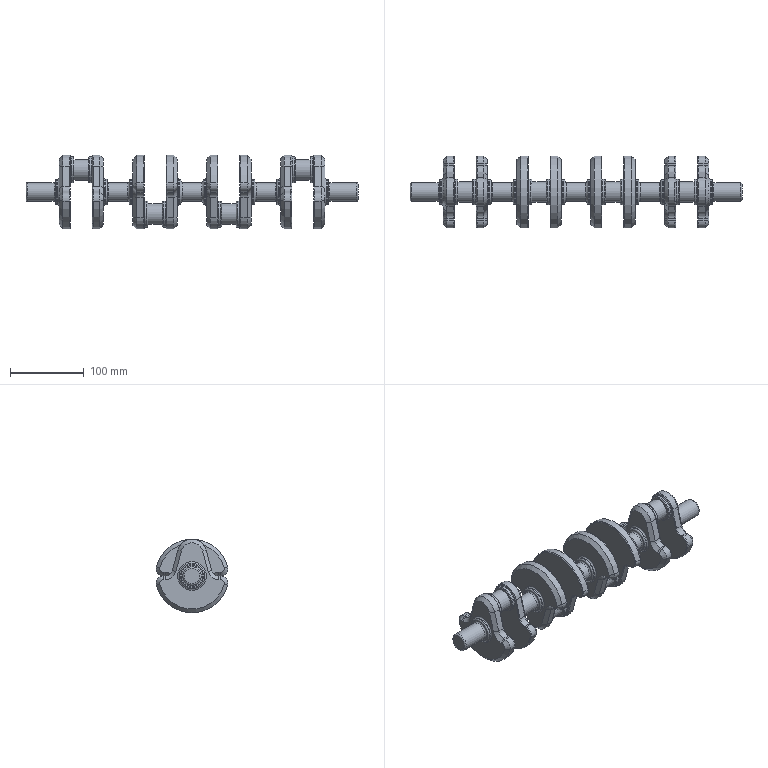Component | NX | CRANK | 1 solid | 341 faces | volume 899987 mm3 | cylinder 105 | plane 98 | torus 90 | cone 48 | commonest cylinder face diameters 20 x32 2 x32 35 x16 100 x8 40 x8 25 x5 28 x4